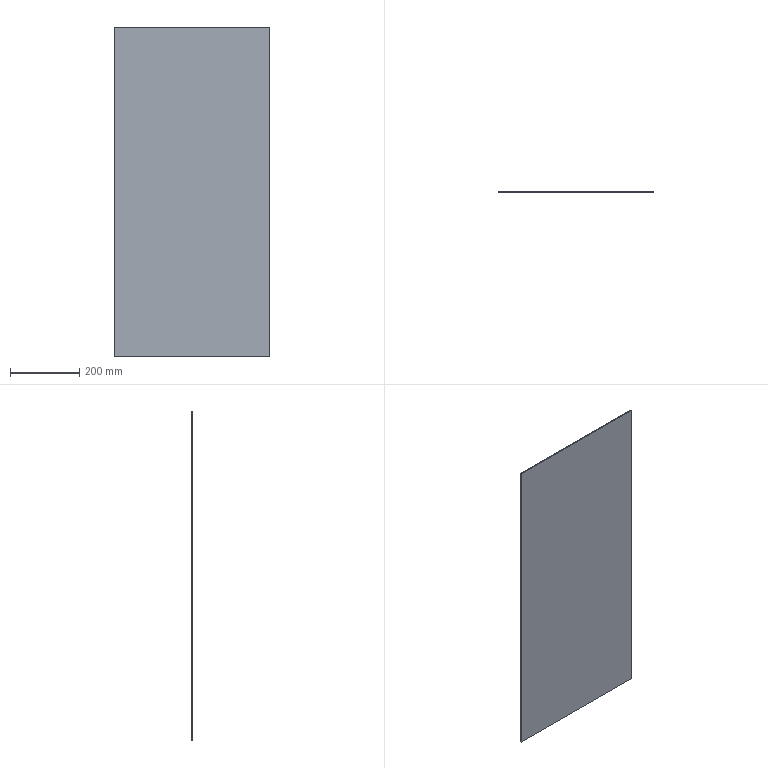Component | SolidWorks | SYM0671-81-101-1_SYM0590-81-103-1 | 1 solid | 6 faces | box 450 x 2 x 950 mm | volume 855000 mm3 | plane 6 | material Plain Carbon Steel
build123d program:
from build123d import *

# Parameters (mm, degrees)
SKETCH1_W      = 450
SKETCH1_H      = 950
EXTRUDE1_DEPTH = 2


with BuildPart() as part:
    # Sketch1 → Extrude1 (new body)
    with BuildSketch(Plane(origin=(0, 0, 0), x_dir=(1, 0, 0), z_dir=(0, 1, 0))):
        with Locations((159.736, -432.667)):
            Rectangle(SKETCH1_W, SKETCH1_H)
    extrude(amount=EXTRUDE1_DEPTH)


solid = part.part

# Placed as in the assembly
solid = solid.moved(Location((-47.485, -478.857, 82.851), (0, 0, 0)))
STEP:
#1=CARTESIAN_POINT('',(-4.439,-18.853,1.595));
#2=VERTEX_POINT('',#1);
#3=CARTESIAN_POINT('',(-4.439,-18.853,38.997));
#4=VERTEX_POINT('',#3);
#5=CARTESIAN_POINT('',(-4.439,-18.853,1.595));
#6=DIRECTION('',(0.,0.,1.));
#7=VECTOR('',#6,39.37);
#8=LINE('',#5,#7);
#9=EDGE_CURVE('',#2,#4,#8,.T.);
#10=ORIENTED_EDGE('',*,*,#9,.T.);
#11=CARTESIAN_POINT('',(-4.439,-18.774,38.997));
#12=VERTEX_POINT('',#11);
#13=CARTESIAN_POINT('',(-4.439,-18.774,38.997));
#14=DIRECTION('',(0.,-1.,0.));
#15=VECTOR('',#14,39.37);
#16=LINE('',#13,#15);
#17=EDGE_CURVE('',#12,#4,#16,.T.);
#18=ORIENTED_EDGE('',*,*,#17,.F.);
#19=CARTESIAN_POINT('',(-4.439,-18.774,1.595));
#20=VERTEX_POINT('',#19);
#21=CARTESIAN_POINT('',(-4.439,-18.774,1.595));
#22=DIRECTION('',(0.,0.,1.));
#23=VECTOR('',#22,39.37);
#24=LINE('',#21,#23);
#25=EDGE_CURVE('',#20,#12,#24,.T.);
#26=ORIENTED_EDGE('',*,*,#25,.F.);
#27=CARTESIAN_POINT('',(-4.439,-18.774,1.595));
#28=DIRECTION('',(0.,-1.,0.));
#29=VECTOR('',#28,39.37);
#30=LINE('',#27,#29);
#31=EDGE_CURVE('',#20,#2,#30,.T.);
#32=ORIENTED_EDGE('',*,*,#31,.T.);
#33=EDGE_LOOP('',(#10,#18,#26,#32));
#34=FACE_OUTER_BOUND('',#33,.T.);
#35=CARTESIAN_POINT('',(-4.439,-18.774,1.595));
#36=DIRECTION('',(1.,0.,-0.));
#37=DIRECTION('',(-0.,0.,-1.));
#38=AXIS2_PLACEMENT_3D('',#35,#36,#37);
#39=PLANE('',#38);
#40=ADVANCED_FACE('',(#34),#39,.F.);
#41=CARTESIAN_POINT('',(13.278,-18.853,38.997));
#42=VERTEX_POINT('',#41);
#43=CARTESIAN_POINT('',(-4.439,-18.853,38.997));
#44=DIRECTION('',(1.,0.,0.));
#45=VECTOR('',#44,39.37);
#46=LINE('',#43,#45);
#47=EDGE_CURVE('',#4,#42,#46,.T.);
#48=ORIENTED_EDGE('',*,*,#47,.T.);
#49=CARTESIAN_POINT('',(13.278,-18.774,38.997));
#50=VERTEX_POINT('',#49);
#51=CARTESIAN_POINT('',(13.278,-18.774,38.997));
#52=DIRECTION('',(0.,-1.,0.));
#53=VECTOR('',#52,39.37);
#54=LINE('',#51,#53);
#55=EDGE_CURVE('',#50,#42,#54,.T.);
#56=ORIENTED_EDGE('',*,*,#55,.F.);
#57=CARTESIAN_POINT('',(-4.439,-18.774,38.997));
#58=DIRECTION('',(1.,0.,0.));
#59=VECTOR('',#58,39.37);
#60=LINE('',#57,#59);
#61=EDGE_CURVE('',#12,#50,#60,.T.);
#62=ORIENTED_EDGE('',*,*,#61,.F.);
#63=ORIENTED_EDGE('',*,*,#17,.T.);
#64=EDGE_LOOP('',(#48,#56,#62,#63));
#65=FACE_OUTER_BOUND('',#64,.T.);
#66=CARTESIAN_POINT('',(-4.439,-18.774,38.997));
#67=DIRECTION('',(0.,0.,-1.));
#68=DIRECTION('',(-1.,0.,0.));
#69=AXIS2_PLACEMENT_3D('',#66,#67,#68);
#70=PLANE('',#69);
#71=ADVANCED_FACE('',(#65),#70,.F.);
#72=CARTESIAN_POINT('',(13.278,-18.853,1.595));
#73=VERTEX_POINT('',#72);
#74=CARTESIAN_POINT('',(13.278,-18.853,1.595));
#75=DIRECTION('',(-0.,0.,-1.));
#76=VECTOR('',#75,39.37);
#77=LINE('',#74,#76);
#78=EDGE_CURVE('',#42,#73,#77,.T.);
#79=ORIENTED_EDGE('',*,*,#78,.T.);
#80=CARTESIAN_POINT('',(13.278,-18.774,1.595));
#81=VERTEX_POINT('',#80);
#82=CARTESIAN_POINT('',(13.278,-18.774,1.595));
#83=DIRECTION('',(0.,-1.,0.));
#84=VECTOR('',#83,39.37);
#85=LINE('',#82,#84);
#86=EDGE_CURVE('',#81,#73,#85,.T.);
#87=ORIENTED_EDGE('',*,*,#86,.F.);
#88=CARTESIAN_POINT('',(13.278,-18.774,1.595));
#89=DIRECTION('',(-0.,0.,-1.));
#90=VECTOR('',#89,39.37);
#91=LINE('',#88,#90);
#92=EDGE_CURVE('',#50,#81,#91,.T.);
#93=ORIENTED_EDGE('',*,*,#92,.F.);
#94=ORIENTED_EDGE('',*,*,#55,.T.);
#95=EDGE_LOOP('',(#79,#87,#93,#94));
#96=FACE_OUTER_BOUND('',#95,.T.);
#97=CARTESIAN_POINT('',(13.278,-18.774,1.595));
#98=DIRECTION('',(-1.,0.,0.));
#99=DIRECTION('',(0.,0.,1.));
#100=AXIS2_PLACEMENT_3D('',#97,#98,#99);
#101=PLANE('',#100);
#102=ADVANCED_FACE('',(#96),#101,.F.);
#103=CARTESIAN_POINT('',(-4.439,-18.853,1.595));
#104=DIRECTION('',(-1.,0.,0.));
#105=VECTOR('',#104,39.37);
#106=LINE('',#103,#105);
#107=EDGE_CURVE('',#73,#2,#106,.T.);
#108=ORIENTED_EDGE('',*,*,#107,.T.);
#109=ORIENTED_EDGE('',*,*,#31,.F.);
#110=CARTESIAN_POINT('',(-4.439,-18.774,1.595));
#111=DIRECTION('',(-1.,0.,0.));
#112=VECTOR('',#111,39.37);
#113=LINE('',#110,#112);
#114=EDGE_CURVE('',#81,#20,#113,.T.);
#115=ORIENTED_EDGE('',*,*,#114,.F.);
#116=ORIENTED_EDGE('',*,*,#86,.T.);
#117=EDGE_LOOP('',(#108,#109,#115,#116));
#118=FACE_OUTER_BOUND('',#117,.T.);
#119=CARTESIAN_POINT('',(-4.439,-18.774,1.595));
#120=DIRECTION('',(0.,0.,1.));
#121=DIRECTION('',(1.,0.,0.));
#122=AXIS2_PLACEMENT_3D('',#119,#120,#121);
#123=PLANE('',#122);
#124=ADVANCED_FACE('',(#118),#123,.F.);
#125=ORIENTED_EDGE('',*,*,#25,.T.);
#126=ORIENTED_EDGE('',*,*,#61,.T.);
#127=ORIENTED_EDGE('',*,*,#92,.T.);
#128=ORIENTED_EDGE('',*,*,#114,.T.);
#129=EDGE_LOOP('',(#125,#126,#127,#128));
#130=FACE_OUTER_BOUND('',#129,.T.);
#131=CARTESIAN_POINT('',(-4.439,-18.774,38.997));
#132=DIRECTION('',(0.,1.,0.));
#133=DIRECTION('',(0.,0.,1.));
#134=AXIS2_PLACEMENT_3D('',#131,#132,#133);
#135=PLANE('',#134);
#136=ADVANCED_FACE('',(#130),#135,.T.);
#137=ORIENTED_EDGE('',*,*,#9,.F.);
#138=ORIENTED_EDGE('',*,*,#107,.F.);
#139=ORIENTED_EDGE('',*,*,#78,.F.);
#140=ORIENTED_EDGE('',*,*,#47,.F.);
#141=EDGE_LOOP('',(#137,#138,#139,#140));
#142=FACE_OUTER_BOUND('',#141,.T.);
#143=CARTESIAN_POINT('',(-4.439,-18.853,38.997));
#144=DIRECTION('',(0.,1.,0.));
#145=DIRECTION('',(0.,0.,1.));
#146=AXIS2_PLACEMENT_3D('',#143,#144,#145);
#147=PLANE('',#146);
#148=ADVANCED_FACE('',(#142),#147,.F.);
#149=CLOSED_SHELL('',(#40,#71,#102,#124,#136,#148));
#150=MANIFOLD_SOLID_BREP('',#149);
#151=CARTESIAN_POINT('',(0.,0.,0.));
#152=DIRECTION('',(0.,0.,1.));
#153=DIRECTION('',(1.,0.,0.));
#154=AXIS2_PLACEMENT_3D('',#151,#152,#153);
#155=(LENGTH_UNIT()NAMED_UNIT(*)SI_UNIT($,.METRE.));
#156=LENGTH_MEASURE_WITH_UNIT(LENGTH_MEASURE(0.0254),#155);
#157=DIMENSIONAL_EXPONENTS(1.,0.,0.,0.,0.,0.,0.);
#158=(CONVERSION_BASED_UNIT('',#156)LENGTH_UNIT()NAMED_UNIT(#157));
#159=UNCERTAINTY_MEASURE_WITH_UNIT(LENGTH_MEASURE(0.00001),#158,'','');
#160=(NAMED_UNIT(*)PLANE_ANGLE_UNIT()SI_UNIT($,.RADIAN.));
#161=(NAMED_UNIT(*)SI_UNIT($,.STERADIAN.)SOLID_ANGLE_UNIT());
#162=(GEOMETRIC_REPRESENTATION_CONTEXT(3)GLOBAL_UNCERTAINTY_ASSIGNED_CONTEXT((#159))GLOBAL_UNIT_ASSIGNED_CONTEXT((#158,#160,#161))REPRESENTATION_CONTEXT('',''));
#163=ADVANCED_BREP_SHAPE_REPRESENTATION('',(#150,#154),#162);
#164=COLOUR_RGB('',0.7922,0.8196,0.9333);
#165=FILL_AREA_STYLE_COLOUR('',#164);
#166=FILL_AREA_STYLE('',(#165));
#167=SURFACE_STYLE_FILL_AREA(#166);
#168=SURFACE_SIDE_STYLE('',(#167));
#169=SURFACE_STYLE_USAGE(.BOTH.,#168);
#170=PRESENTATION_STYLE_ASSIGNMENT((#169));
#171=STYLED_ITEM('',(#170),#150);
#172=(LENGTH_UNIT()NAMED_UNIT(*)SI_UNIT($,.METRE.));
#173=LENGTH_MEASURE_WITH_UNIT(LENGTH_MEASURE(0.0254),#172);
#174=DIMENSIONAL_EXPONENTS(1.,0.,0.,0.,0.,0.,0.);
#175=(CONVERSION_BASED_UNIT('',#173)LENGTH_UNIT()NAMED_UNIT(#174));
#176=UNCERTAINTY_MEASURE_WITH_UNIT(LENGTH_MEASURE(0.00001),#175,'','');
#177=(NAMED_UNIT(*)PLANE_ANGLE_UNIT()SI_UNIT($,.RADIAN.));
#178=(NAMED_UNIT(*)SI_UNIT($,.STERADIAN.)SOLID_ANGLE_UNIT());
#179=(GEOMETRIC_REPRESENTATION_CONTEXT(3)GLOBAL_UNCERTAINTY_ASSIGNED_CONTEXT((#176))GLOBAL_UNIT_ASSIGNED_CONTEXT((#175,#177,#178))REPRESENTATION_CONTEXT('',''));
#180=MECHANICAL_DESIGN_GEOMETRIC_PRESENTATION_REPRESENTATION('',(#171),#179);
#181=PRESENTATION_LAYER_ASSIGNMENT('','',(#171));